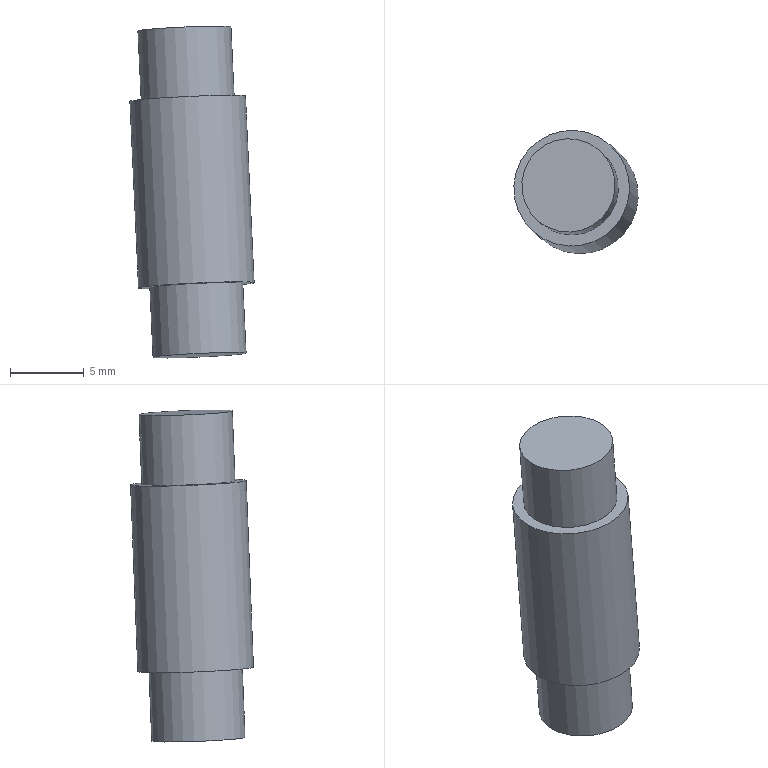Component | NX | PASADOR_B | 1 solid | 7 faces | box 8.45 x 8.36 x 22.57 mm | volume 920 mm3 | plane 4 | cylinder 3 | commonest cylinder face diameters 6.35 x2 7.874 x1
STEP:
#1=CARTESIAN_POINT('',(0.,0.,0.));
#2=DIRECTION('',(0.,0.,1.));
#3=DIRECTION('',(1.,0.,0.));
#4=AXIS2_PLACEMENT_3D('',#1,#2,#3);
#5=CARTESIAN_POINT('',(61.3,9.067,12.132));
#6=VERTEX_POINT('',#5);
#7=CARTESIAN_POINT('',(64.928,10.592,12.241));
#8=DIRECTION('',(0.04625,-0.03881,-0.9982));
#9=DIRECTION('',(-0.9215,-0.3874,-0.02763));
#10=AXIS2_PLACEMENT_3D('',#7,#8,#9);
#11=CIRCLE('',#10,3.937);
#12=CARTESIAN_POINT('',(64.928,10.592,12.241));
#13=DIRECTION('',(0.04625,-0.03881,-0.9982));
#14=DIRECTION('',(-0.9215,-0.3874,-0.02763));
#15=AXIS2_PLACEMENT_3D('',#12,#13,#14);
#16=CYLINDRICAL_SURFACE('',#15,3.937);
#17=CARTESIAN_POINT('',(0.,0.));
#18=DIRECTION('',(1.,0.));
#19=VECTOR('',#18,1.);
#20=LINE('',#17,#19);
#21=(GEOMETRIC_REPRESENTATION_CONTEXT(2)PARAMETRIC_REPRESENTATION_CONTEXT()REPRESENTATION_CONTEXT('',''));
#22=DEFINITIONAL_REPRESENTATION('',(#20),#21);
#23=PCURVE('',#16,#22);
#24=CARTESIAN_POINT('',(64.928,10.592,12.241));
#25=DIRECTION('',(0.04625,-0.03881,-0.9982));
#26=DIRECTION('',(-0.9215,-0.3874,-0.02763));
#27=AXIS2_PLACEMENT_3D('',#24,#25,#26);
#28=PLANE('',#27);
#29=CARTESIAN_POINT('',(0.,0.));
#30=DIRECTION('',(1.,-0.));
#31=AXIS2_PLACEMENT_2D('',#29,#30);
#32=CIRCLE('',#31,3.937);
#33=(GEOMETRIC_REPRESENTATION_CONTEXT(2)PARAMETRIC_REPRESENTATION_CONTEXT()REPRESENTATION_CONTEXT('',''));
#34=DEFINITIONAL_REPRESENTATION('',(#32),#33);
#35=PCURVE('',#28,#34);
#36=SURFACE_CURVE('',#11,(#23,#35),.PCURVE_S1.);
#37=EDGE_CURVE('',#6,#6,#36,.T.);
#38=ORIENTED_EDGE('',*,*,#37,.T.);
#39=CARTESIAN_POINT('',(61.888,8.574,-0.5444));
#40=VERTEX_POINT('',#39);
#41=CARTESIAN_POINT('',(61.3,9.067,12.132));
#42=CARTESIAN_POINT('',(61.888,8.574,-0.5444));
#43=B_SPLINE_CURVE_WITH_KNOTS('',1,(#41,#42),.UNSPECIFIED.,.F.,.F.,(2,2),(0.,12.7),.PIECEWISE_BEZIER_KNOTS.);
#44=CARTESIAN_POINT('',(6.283,0.));
#45=DIRECTION('',(0.,1.));
#46=VECTOR('',#45,1.);
#47=LINE('',#44,#46);
#48=(GEOMETRIC_REPRESENTATION_CONTEXT(2)PARAMETRIC_REPRESENTATION_CONTEXT()REPRESENTATION_CONTEXT('',''));
#49=DEFINITIONAL_REPRESENTATION('',(#47),#48);
#50=PCURVE('',#16,#49);
#51=CARTESIAN_POINT('',(0.,0.));
#52=DIRECTION('',(0.,1.));
#53=VECTOR('',#52,1.);
#54=LINE('',#51,#53);
#55=(GEOMETRIC_REPRESENTATION_CONTEXT(2)PARAMETRIC_REPRESENTATION_CONTEXT()REPRESENTATION_CONTEXT('',''));
#56=DEFINITIONAL_REPRESENTATION('',(#54),#55);
#57=PCURVE('',#16,#56);
#58=SEAM_CURVE('',#43,(#50,#57),.PCURVE_S1.);
#59=EDGE_CURVE('',#6,#40,#58,.T.);
#60=ORIENTED_EDGE('',*,*,#59,.T.);
#61=CARTESIAN_POINT('',(65.515,10.1,-0.4356));
#62=DIRECTION('',(0.04625,-0.03881,-0.9982));
#63=DIRECTION('',(-0.9215,-0.3874,-0.02763));
#64=AXIS2_PLACEMENT_3D('',#61,#62,#63);
#65=CIRCLE('',#64,3.937);
#66=CARTESIAN_POINT('',(0.,12.7));
#67=DIRECTION('',(1.,0.));
#68=VECTOR('',#67,1.);
#69=LINE('',#66,#68);
#70=(GEOMETRIC_REPRESENTATION_CONTEXT(2)PARAMETRIC_REPRESENTATION_CONTEXT()REPRESENTATION_CONTEXT('',''));
#71=DEFINITIONAL_REPRESENTATION('',(#69),#70);
#72=PCURVE('',#16,#71);
#73=CARTESIAN_POINT('',(65.515,10.1,-0.4356));
#74=DIRECTION('',(0.04625,-0.03881,-0.9982));
#75=DIRECTION('',(-0.9215,-0.3874,-0.02763));
#76=AXIS2_PLACEMENT_3D('',#73,#74,#75);
#77=PLANE('',#76);
#78=CARTESIAN_POINT('',(0.,0.));
#79=DIRECTION('',(1.,-0.));
#80=AXIS2_PLACEMENT_2D('',#78,#79);
#81=CIRCLE('',#80,3.937);
#82=(GEOMETRIC_REPRESENTATION_CONTEXT(2)PARAMETRIC_REPRESENTATION_CONTEXT()REPRESENTATION_CONTEXT('',''));
#83=DEFINITIONAL_REPRESENTATION('',(#81),#82);
#84=PCURVE('',#77,#83);
#85=SURFACE_CURVE('',#65,(#72,#84),.PCURVE_S1.);
#86=EDGE_CURVE('',#40,#40,#85,.T.);
#87=ORIENTED_EDGE('',*,*,#86,.F.);
#88=ORIENTED_EDGE('',*,*,#59,.F.);
#89=EDGE_LOOP('',(#38,#60,#87,#88));
#90=FACE_BOUND('',#89,.T.);
#91=ADVANCED_FACE('',(#90),#16,.T.);
#92=CARTESIAN_POINT('',(62.002,9.363,12.154));
#93=VERTEX_POINT('',#92);
#94=CARTESIAN_POINT('',(64.928,10.592,12.241));
#95=DIRECTION('',(0.04625,-0.03881,-0.9982));
#96=DIRECTION('',(-0.9215,-0.3874,-0.02763));
#97=AXIS2_PLACEMENT_3D('',#94,#95,#96);
#98=CIRCLE('',#97,3.175);
#99=CARTESIAN_POINT('',(0.,0.));
#100=DIRECTION('',(1.,-0.));
#101=AXIS2_PLACEMENT_2D('',#99,#100);
#102=CIRCLE('',#101,3.175);
#103=(GEOMETRIC_REPRESENTATION_CONTEXT(2)PARAMETRIC_REPRESENTATION_CONTEXT()REPRESENTATION_CONTEXT('',''));
#104=DEFINITIONAL_REPRESENTATION('',(#102),#103);
#105=PCURVE('',#28,#104);
#106=CARTESIAN_POINT('',(64.708,10.777,16.995));
#107=DIRECTION('',(0.04625,-0.03881,-0.9982));
#108=DIRECTION('',(-0.9215,-0.3874,-0.02763));
#109=AXIS2_PLACEMENT_3D('',#106,#107,#108);
#110=CYLINDRICAL_SURFACE('',#109,3.175);
#111=CARTESIAN_POINT('',(0.,4.763));
#112=DIRECTION('',(1.,0.));
#113=VECTOR('',#112,1.);
#114=LINE('',#111,#113);
#115=(GEOMETRIC_REPRESENTATION_CONTEXT(2)PARAMETRIC_REPRESENTATION_CONTEXT()REPRESENTATION_CONTEXT('',''));
#116=DEFINITIONAL_REPRESENTATION('',(#114),#115);
#117=PCURVE('',#110,#116);
#118=SURFACE_CURVE('',#98,(#105,#117),.PCURVE_S1.);
#119=EDGE_CURVE('',#93,#93,#118,.T.);
#120=ORIENTED_EDGE('',*,*,#119,.T.);
#121=EDGE_LOOP('',(#120));
#122=FACE_BOUND('',#121,.T.);
#123=ORIENTED_EDGE('',*,*,#37,.F.);
#124=EDGE_LOOP('',(#123));
#125=FACE_BOUND('',#124,.T.);
#126=ADVANCED_FACE('',(#122,#125),#28,.F.);
#127=CARTESIAN_POINT('',(62.59,8.87,-0.5233));
#128=VERTEX_POINT('',#127);
#129=CARTESIAN_POINT('',(65.515,10.1,-0.4356));
#130=DIRECTION('',(0.04625,-0.03881,-0.9982));
#131=DIRECTION('',(-0.9215,-0.3874,-0.02763));
#132=AXIS2_PLACEMENT_3D('',#129,#130,#131);
#133=CIRCLE('',#132,3.175);
#134=CARTESIAN_POINT('',(0.,0.));
#135=DIRECTION('',(1.,-0.));
#136=AXIS2_PLACEMENT_2D('',#134,#135);
#137=CIRCLE('',#136,3.175);
#138=(GEOMETRIC_REPRESENTATION_CONTEXT(2)PARAMETRIC_REPRESENTATION_CONTEXT()REPRESENTATION_CONTEXT('',''));
#139=DEFINITIONAL_REPRESENTATION('',(#137),#138);
#140=PCURVE('',#77,#139);
#141=CARTESIAN_POINT('',(64.708,10.777,16.995));
#142=DIRECTION('',(0.04625,-0.03881,-0.9982));
#143=DIRECTION('',(-0.9215,-0.3874,-0.02763));
#144=AXIS2_PLACEMENT_3D('',#141,#142,#143);
#145=CYLINDRICAL_SURFACE('',#144,3.175);
#146=CARTESIAN_POINT('',(0.,17.462));
#147=DIRECTION('',(1.,0.));
#148=VECTOR('',#147,1.);
#149=LINE('',#146,#148);
#150=(GEOMETRIC_REPRESENTATION_CONTEXT(2)PARAMETRIC_REPRESENTATION_CONTEXT()REPRESENTATION_CONTEXT('',''));
#151=DEFINITIONAL_REPRESENTATION('',(#149),#150);
#152=PCURVE('',#145,#151);
#153=SURFACE_CURVE('',#133,(#140,#152),.PCURVE_S1.);
#154=EDGE_CURVE('',#128,#128,#153,.T.);
#155=ORIENTED_EDGE('',*,*,#154,.F.);
#156=EDGE_LOOP('',(#155));
#157=FACE_BOUND('',#156,.T.);
#158=ORIENTED_EDGE('',*,*,#86,.T.);
#159=EDGE_LOOP('',(#158));
#160=FACE_BOUND('',#159,.T.);
#161=ADVANCED_FACE('',(#157,#160),#77,.T.);
#162=CARTESIAN_POINT('',(62.81,8.685,-5.277));
#163=VERTEX_POINT('',#162);
#164=CARTESIAN_POINT('',(65.736,9.915,-5.189));
#165=DIRECTION('',(0.04625,-0.03881,-0.9982));
#166=DIRECTION('',(-0.9215,-0.3874,-0.02763));
#167=AXIS2_PLACEMENT_3D('',#164,#165,#166);
#168=CIRCLE('',#167,3.175);
#169=CARTESIAN_POINT('',(65.736,9.915,-5.189));
#170=DIRECTION('',(0.04625,-0.03881,-0.9982));
#171=DIRECTION('',(-0.9215,-0.3874,-0.02763));
#172=AXIS2_PLACEMENT_3D('',#169,#170,#171);
#173=PLANE('',#172);
#174=CARTESIAN_POINT('',(0.,0.));
#175=DIRECTION('',(1.,-0.));
#176=AXIS2_PLACEMENT_2D('',#174,#175);
#177=CIRCLE('',#176,3.175);
#178=(GEOMETRIC_REPRESENTATION_CONTEXT(2)PARAMETRIC_REPRESENTATION_CONTEXT()REPRESENTATION_CONTEXT('',''));
#179=DEFINITIONAL_REPRESENTATION('',(#177),#178);
#180=PCURVE('',#173,#179);
#181=CARTESIAN_POINT('',(0.,22.225));
#182=DIRECTION('',(1.,0.));
#183=VECTOR('',#182,1.);
#184=LINE('',#181,#183);
#185=(GEOMETRIC_REPRESENTATION_CONTEXT(2)PARAMETRIC_REPRESENTATION_CONTEXT()REPRESENTATION_CONTEXT('',''));
#186=DEFINITIONAL_REPRESENTATION('',(#184),#185);
#187=PCURVE('',#145,#186);
#188=SURFACE_CURVE('',#168,(#180,#187),.PCURVE_S1.);
#189=EDGE_CURVE('',#163,#163,#188,.T.);
#190=ORIENTED_EDGE('',*,*,#189,.T.);
#191=EDGE_LOOP('',(#190));
#192=FACE_BOUND('',#191,.T.);
#193=ADVANCED_FACE('',(#192),#173,.T.);
#194=ORIENTED_EDGE('',*,*,#154,.T.);
#195=CARTESIAN_POINT('',(62.59,8.87,-0.5233));
#196=CARTESIAN_POINT('',(62.81,8.685,-5.277));
#197=B_SPLINE_CURVE_WITH_KNOTS('',1,(#195,#196),.UNSPECIFIED.,.F.,.F.,(2,2),(17.462,22.225),.PIECEWISE_BEZIER_KNOTS.);
#198=CARTESIAN_POINT('',(6.283,0.));
#199=DIRECTION('',(0.,1.));
#200=VECTOR('',#199,1.);
#201=LINE('',#198,#200);
#202=(GEOMETRIC_REPRESENTATION_CONTEXT(2)PARAMETRIC_REPRESENTATION_CONTEXT()REPRESENTATION_CONTEXT('',''));
#203=DEFINITIONAL_REPRESENTATION('',(#201),#202);
#204=PCURVE('',#145,#203);
#205=CARTESIAN_POINT('',(0.,0.));
#206=DIRECTION('',(0.,1.));
#207=VECTOR('',#206,1.);
#208=LINE('',#205,#207);
#209=(GEOMETRIC_REPRESENTATION_CONTEXT(2)PARAMETRIC_REPRESENTATION_CONTEXT()REPRESENTATION_CONTEXT('',''));
#210=DEFINITIONAL_REPRESENTATION('',(#208),#209);
#211=PCURVE('',#145,#210);
#212=SEAM_CURVE('',#197,(#204,#211),.PCURVE_S1.);
#213=EDGE_CURVE('',#128,#163,#212,.T.);
#214=ORIENTED_EDGE('',*,*,#213,.T.);
#215=ORIENTED_EDGE('',*,*,#189,.F.);
#216=ORIENTED_EDGE('',*,*,#213,.F.);
#217=EDGE_LOOP('',(#194,#214,#215,#216));
#218=FACE_BOUND('',#217,.T.);
#219=ADVANCED_FACE('',(#218),#145,.T.);
#220=CARTESIAN_POINT('',(61.782,9.547,16.907));
#221=VERTEX_POINT('',#220);
#222=CARTESIAN_POINT('',(64.708,10.777,16.995));
#223=DIRECTION('',(0.04625,-0.03881,-0.9982));
#224=DIRECTION('',(-0.9215,-0.3874,-0.02763));
#225=AXIS2_PLACEMENT_3D('',#222,#223,#224);
#226=CIRCLE('',#225,3.175);
#227=CARTESIAN_POINT('',(0.,0.));
#228=DIRECTION('',(1.,0.));
#229=VECTOR('',#228,1.);
#230=LINE('',#227,#229);
#231=(GEOMETRIC_REPRESENTATION_CONTEXT(2)PARAMETRIC_REPRESENTATION_CONTEXT()REPRESENTATION_CONTEXT('',''));
#232=DEFINITIONAL_REPRESENTATION('',(#230),#231);
#233=PCURVE('',#110,#232);
#234=CARTESIAN_POINT('',(64.708,10.777,16.995));
#235=DIRECTION('',(0.04625,-0.03881,-0.9982));
#236=DIRECTION('',(-0.9215,-0.3874,-0.02763));
#237=AXIS2_PLACEMENT_3D('',#234,#235,#236);
#238=PLANE('',#237);
#239=CARTESIAN_POINT('',(0.,0.));
#240=DIRECTION('',(1.,-0.));
#241=AXIS2_PLACEMENT_2D('',#239,#240);
#242=CIRCLE('',#241,3.175);
#243=(GEOMETRIC_REPRESENTATION_CONTEXT(2)PARAMETRIC_REPRESENTATION_CONTEXT()REPRESENTATION_CONTEXT('',''));
#244=DEFINITIONAL_REPRESENTATION('',(#242),#243);
#245=PCURVE('',#238,#244);
#246=SURFACE_CURVE('',#226,(#233,#245),.PCURVE_S1.);
#247=EDGE_CURVE('',#221,#221,#246,.T.);
#248=ORIENTED_EDGE('',*,*,#247,.T.);
#249=CARTESIAN_POINT('',(61.782,9.547,16.907));
#250=CARTESIAN_POINT('',(62.002,9.363,12.154));
#251=B_SPLINE_CURVE_WITH_KNOTS('',1,(#249,#250),.UNSPECIFIED.,.F.,.F.,(2,2),(0.,4.763),.PIECEWISE_BEZIER_KNOTS.);
#252=CARTESIAN_POINT('',(6.283,0.));
#253=DIRECTION('',(0.,1.));
#254=VECTOR('',#253,1.);
#255=LINE('',#252,#254);
#256=(GEOMETRIC_REPRESENTATION_CONTEXT(2)PARAMETRIC_REPRESENTATION_CONTEXT()REPRESENTATION_CONTEXT('',''));
#257=DEFINITIONAL_REPRESENTATION('',(#255),#256);
#258=PCURVE('',#110,#257);
#259=CARTESIAN_POINT('',(0.,0.));
#260=DIRECTION('',(0.,1.));
#261=VECTOR('',#260,1.);
#262=LINE('',#259,#261);
#263=(GEOMETRIC_REPRESENTATION_CONTEXT(2)PARAMETRIC_REPRESENTATION_CONTEXT()REPRESENTATION_CONTEXT('',''));
#264=DEFINITIONAL_REPRESENTATION('',(#262),#263);
#265=PCURVE('',#110,#264);
#266=SEAM_CURVE('',#251,(#258,#265),.PCURVE_S1.);
#267=EDGE_CURVE('',#221,#93,#266,.T.);
#268=ORIENTED_EDGE('',*,*,#267,.T.);
#269=ORIENTED_EDGE('',*,*,#119,.F.);
#270=ORIENTED_EDGE('',*,*,#267,.F.);
#271=EDGE_LOOP('',(#248,#268,#269,#270));
#272=FACE_BOUND('',#271,.T.);
#273=ADVANCED_FACE('',(#272),#110,.T.);
#274=ORIENTED_EDGE('',*,*,#247,.F.);
#275=EDGE_LOOP('',(#274));
#276=FACE_BOUND('',#275,.T.);
#277=ADVANCED_FACE('',(#276),#238,.F.);
#278=CLOSED_SHELL('',(#91,#126,#161,#193,#219,#273,#277));
#279=MANIFOLD_SOLID_BREP('',#278);
#280=(LENGTH_UNIT()NAMED_UNIT(*)SI_UNIT(.MILLI.,.METRE.));
#281=UNCERTAINTY_MEASURE_WITH_UNIT(LENGTH_MEASURE(0.00001),#280,'','');
#282=(NAMED_UNIT(*)PLANE_ANGLE_UNIT()SI_UNIT($,.RADIAN.));
#283=(NAMED_UNIT(*)SI_UNIT($,.STERADIAN.)SOLID_ANGLE_UNIT());
#284=(GEOMETRIC_REPRESENTATION_CONTEXT(3)GLOBAL_UNCERTAINTY_ASSIGNED_CONTEXT((#281))GLOBAL_UNIT_ASSIGNED_CONTEXT((#280,#282,#283))REPRESENTATION_CONTEXT('',''));
#285=ADVANCED_BREP_SHAPE_REPRESENTATION('',(#4,#279),#284);